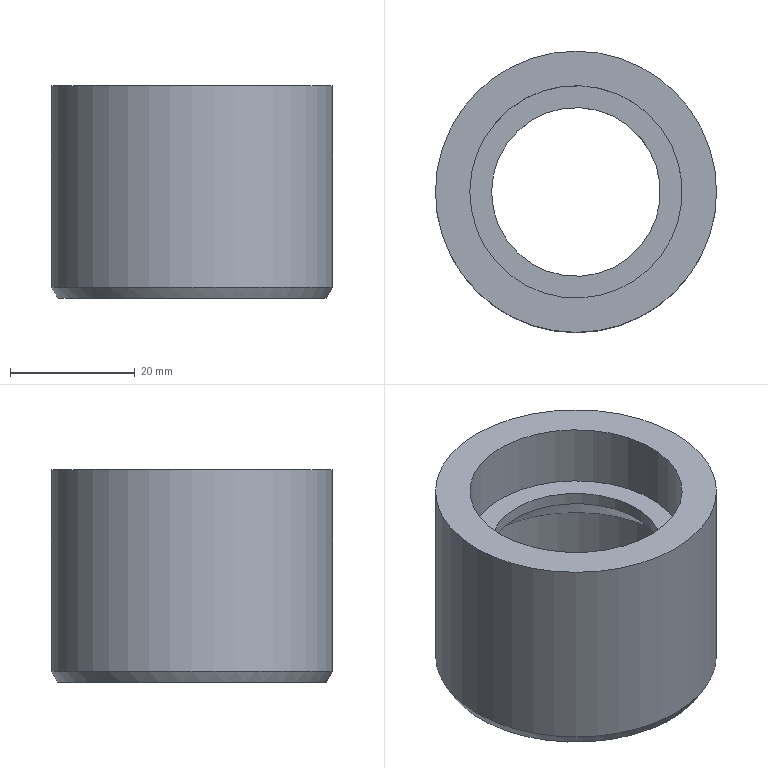Component | NX | CH3404_8_1-1 | 1 solid | 9 faces | box 45 x 45 x 34 mm | volume 19820 mm3 | cylinder 4 | plane 3 | cone 2 | commonest cylinder face diameters 45 x1 38.6 x1 27 x1 34 x1
STEP:
#1=CARTESIAN_POINT('',(0.,0.,0.));
#2=DIRECTION('',(0.,0.,1.));
#3=DIRECTION('',(1.,0.,0.));
#4=AXIS2_PLACEMENT_3D('',#1,#2,#3);
#5=CARTESIAN_POINT('',(-22.5,0.,137.));
#6=VERTEX_POINT('',#5);
#7=CARTESIAN_POINT('',(0.,0.,137.));
#8=DIRECTION('',(0.,0.,-1.));
#9=DIRECTION('',(-1.,0.,0.));
#10=AXIS2_PLACEMENT_3D('',#7,#8,#9);
#11=CIRCLE('',#10,22.5);
#12=CARTESIAN_POINT('',(0.,-17.,137.));
#13=DIRECTION('',(0.,0.,-1.));
#14=DIRECTION('',(-1.,0.,0.));
#15=AXIS2_PLACEMENT_3D('',#12,#13,#14);
#16=PLANE('',#15);
#17=CARTESIAN_POINT('',(0.,17.));
#18=DIRECTION('',(1.,0.));
#19=AXIS2_PLACEMENT_2D('',#17,#18);
#20=CIRCLE('',#19,22.5);
#21=(GEOMETRIC_REPRESENTATION_CONTEXT(2)PARAMETRIC_REPRESENTATION_CONTEXT()REPRESENTATION_CONTEXT('',''));
#22=DEFINITIONAL_REPRESENTATION('',(#20),#21);
#23=PCURVE('',#16,#22);
#24=CARTESIAN_POINT('',(0.,0.,103.));
#25=DIRECTION('',(0.,0.,-1.));
#26=DIRECTION('',(-1.,0.,0.));
#27=AXIS2_PLACEMENT_3D('',#24,#25,#26);
#28=CYLINDRICAL_SURFACE('',#27,22.5);
#29=CARTESIAN_POINT('',(0.,-34.));
#30=DIRECTION('',(1.,0.));
#31=VECTOR('',#30,1.);
#32=LINE('',#29,#31);
#33=(GEOMETRIC_REPRESENTATION_CONTEXT(2)PARAMETRIC_REPRESENTATION_CONTEXT()REPRESENTATION_CONTEXT('',''));
#34=DEFINITIONAL_REPRESENTATION('',(#32),#33);
#35=PCURVE('',#28,#34);
#36=SURFACE_CURVE('',#11,(#23,#35),.PCURVE_S1.);
#37=EDGE_CURVE('',#6,#6,#36,.T.);
#38=ORIENTED_EDGE('',*,*,#37,.F.);
#39=EDGE_LOOP('',(#38));
#40=FACE_BOUND('',#39,.T.);
#41=CARTESIAN_POINT('',(-17.,0.,137.));
#42=VERTEX_POINT('',#41);
#43=CARTESIAN_POINT('',(0.,0.,137.));
#44=DIRECTION('',(0.,0.,-1.));
#45=DIRECTION('',(-1.,0.,0.));
#46=AXIS2_PLACEMENT_3D('',#43,#44,#45);
#47=CIRCLE('',#46,17.);
#48=CARTESIAN_POINT('',(0.,17.));
#49=DIRECTION('',(1.,0.));
#50=AXIS2_PLACEMENT_2D('',#48,#49);
#51=CIRCLE('',#50,17.);
#52=(GEOMETRIC_REPRESENTATION_CONTEXT(2)PARAMETRIC_REPRESENTATION_CONTEXT()REPRESENTATION_CONTEXT('',''));
#53=DEFINITIONAL_REPRESENTATION('',(#51),#52);
#54=PCURVE('',#16,#53);
#55=CARTESIAN_POINT('',(0.,0.,103.));
#56=DIRECTION('',(0.,0.,-1.));
#57=DIRECTION('',(-1.,0.,0.));
#58=AXIS2_PLACEMENT_3D('',#55,#56,#57);
#59=CYLINDRICAL_SURFACE('',#58,17.);
#60=CARTESIAN_POINT('',(0.,-34.));
#61=DIRECTION('',(1.,0.));
#62=VECTOR('',#61,1.);
#63=LINE('',#60,#62);
#64=(GEOMETRIC_REPRESENTATION_CONTEXT(2)PARAMETRIC_REPRESENTATION_CONTEXT()REPRESENTATION_CONTEXT('',''));
#65=DEFINITIONAL_REPRESENTATION('',(#63),#64);
#66=PCURVE('',#59,#65);
#67=SURFACE_CURVE('',#47,(#54,#66),.PCURVE_S1.);
#68=EDGE_CURVE('',#42,#42,#67,.T.);
#69=ORIENTED_EDGE('',*,*,#68,.T.);
#70=EDGE_LOOP('',(#69));
#71=FACE_BOUND('',#70,.T.);
#72=ADVANCED_FACE('',(#40,#71),#16,.F.);
#73=CARTESIAN_POINT('',(22.5,0.,104.732));
#74=VERTEX_POINT('',#73);
#75=CARTESIAN_POINT('',(-22.5,0.,104.732));
#76=VERTEX_POINT('',#75);
#77=CARTESIAN_POINT('',(0.,0.,104.732));
#78=DIRECTION('',(0.,0.,1.));
#79=DIRECTION('',(1.,0.,0.));
#80=AXIS2_PLACEMENT_3D('',#77,#78,#79);
#81=CIRCLE('',#80,22.5);
#82=CARTESIAN_POINT('',(3.142,-1.732));
#83=DIRECTION('',(-1.,0.));
#84=VECTOR('',#83,1.);
#85=LINE('',#82,#84);
#86=(GEOMETRIC_REPRESENTATION_CONTEXT(2)PARAMETRIC_REPRESENTATION_CONTEXT()REPRESENTATION_CONTEXT('',''));
#87=DEFINITIONAL_REPRESENTATION('',(#85),#86);
#88=PCURVE('',#28,#87);
#89=CARTESIAN_POINT('',(0.,0.,103.));
#90=DIRECTION('',(0.,0.,1.));
#91=DIRECTION('',(1.,0.,0.));
#92=AXIS2_PLACEMENT_3D('',#89,#90,#91);
#93=CONICAL_SURFACE('',#92,21.5,0.5236);
#94=CARTESIAN_POINT('',(0.,1.732));
#95=DIRECTION('',(1.,0.));
#96=VECTOR('',#95,1.);
#97=LINE('',#94,#96);
#98=(GEOMETRIC_REPRESENTATION_CONTEXT(2)PARAMETRIC_REPRESENTATION_CONTEXT()REPRESENTATION_CONTEXT('',''));
#99=DEFINITIONAL_REPRESENTATION('',(#97),#98);
#100=PCURVE('',#93,#99);
#101=SURFACE_CURVE('',#81,(#88,#100),.PCURVE_S1.);
#102=EDGE_CURVE('',#74,#76,#101,.T.);
#103=ORIENTED_EDGE('',*,*,#102,.T.);
#104=CARTESIAN_POINT('',(-22.5,-0.,137.));
#105=CARTESIAN_POINT('',(-22.5,-0.,104.732));
#106=B_SPLINE_CURVE_WITH_KNOTS('',1,(#104,#105),.UNSPECIFIED.,.F.,.F.,(2,2),(-34.,-1.732),.PIECEWISE_BEZIER_KNOTS.);
#107=CARTESIAN_POINT('',(0.,0.));
#108=DIRECTION('',(0.,1.));
#109=VECTOR('',#108,1.);
#110=LINE('',#107,#109);
#111=(GEOMETRIC_REPRESENTATION_CONTEXT(2)PARAMETRIC_REPRESENTATION_CONTEXT()REPRESENTATION_CONTEXT('',''));
#112=DEFINITIONAL_REPRESENTATION('',(#110),#111);
#113=PCURVE('',#28,#112);
#114=CARTESIAN_POINT('',(6.283,0.));
#115=DIRECTION('',(0.,1.));
#116=VECTOR('',#115,1.);
#117=LINE('',#114,#116);
#118=(GEOMETRIC_REPRESENTATION_CONTEXT(2)PARAMETRIC_REPRESENTATION_CONTEXT()REPRESENTATION_CONTEXT('',''));
#119=DEFINITIONAL_REPRESENTATION('',(#117),#118);
#120=PCURVE('',#28,#119);
#121=SEAM_CURVE('',#106,(#113,#120),.PCURVE_S1.);
#122=EDGE_CURVE('',#6,#76,#121,.T.);
#123=ORIENTED_EDGE('',*,*,#122,.F.);
#124=ORIENTED_EDGE('',*,*,#37,.T.);
#125=ORIENTED_EDGE('',*,*,#122,.T.);
#126=CARTESIAN_POINT('',(0.,0.,104.732));
#127=DIRECTION('',(0.,0.,1.));
#128=DIRECTION('',(1.,0.,0.));
#129=AXIS2_PLACEMENT_3D('',#126,#127,#128);
#130=CIRCLE('',#129,22.5);
#131=CARTESIAN_POINT('',(9.425,-1.732));
#132=DIRECTION('',(-1.,0.));
#133=VECTOR('',#132,1.);
#134=LINE('',#131,#133);
#135=(GEOMETRIC_REPRESENTATION_CONTEXT(2)PARAMETRIC_REPRESENTATION_CONTEXT()REPRESENTATION_CONTEXT('',''));
#136=DEFINITIONAL_REPRESENTATION('',(#134),#135);
#137=PCURVE('',#28,#136);
#138=CARTESIAN_POINT('',(0.,1.732));
#139=DIRECTION('',(1.,0.));
#140=VECTOR('',#139,1.);
#141=LINE('',#138,#140);
#142=(GEOMETRIC_REPRESENTATION_CONTEXT(2)PARAMETRIC_REPRESENTATION_CONTEXT()REPRESENTATION_CONTEXT('',''));
#143=DEFINITIONAL_REPRESENTATION('',(#141),#142);
#144=PCURVE('',#93,#143);
#145=SURFACE_CURVE('',#130,(#137,#144),.PCURVE_S1.);
#146=EDGE_CURVE('',#76,#74,#145,.T.);
#147=ORIENTED_EDGE('',*,*,#146,.T.);
#148=EDGE_LOOP('',(#103,#123,#124,#125,#147));
#149=FACE_BOUND('',#148,.T.);
#150=ADVANCED_FACE('',(#149),#28,.T.);
#151=CARTESIAN_POINT('',(21.5,0.,103.));
#152=VERTEX_POINT('',#151);
#153=CARTESIAN_POINT('',(0.,0.,103.));
#154=DIRECTION('',(0.,0.,-1.));
#155=DIRECTION('',(1.,0.,0.));
#156=AXIS2_PLACEMENT_3D('',#153,#154,#155);
#157=CIRCLE('',#156,21.5);
#158=CARTESIAN_POINT('',(0.,-22.5,103.));
#159=DIRECTION('',(0.,0.,1.));
#160=DIRECTION('',(1.,0.,0.));
#161=AXIS2_PLACEMENT_3D('',#158,#159,#160);
#162=PLANE('',#161);
#163=CARTESIAN_POINT('',(21.5,22.5));
#164=CARTESIAN_POINT('',(21.5,-14.739));
#165=CARTESIAN_POINT('',(-10.75,3.88));
#166=CARTESIAN_POINT('',(-43.,22.5));
#167=CARTESIAN_POINT('',(-10.75,41.12));
#168=CARTESIAN_POINT('',(21.5,59.739));
#169=CARTESIAN_POINT('',(21.5,22.5));
#170=(BOUNDED_CURVE()B_SPLINE_CURVE(2,(#163,#164,#165,#166,#167,#168,#169),.UNSPECIFIED.,.T.,.F.)B_SPLINE_CURVE_WITH_KNOTS((1,2,2,2,2,1),(-2.094,0.,2.094,4.189,6.283,8.378),.UNSPECIFIED.)CURVE()GEOMETRIC_REPRESENTATION_ITEM()RATIONAL_B_SPLINE_CURVE((1.,0.5,1.,0.5,1.,0.5,1.))REPRESENTATION_ITEM(''));
#171=(GEOMETRIC_REPRESENTATION_CONTEXT(2)PARAMETRIC_REPRESENTATION_CONTEXT()REPRESENTATION_CONTEXT('',''));
#172=DEFINITIONAL_REPRESENTATION('',(#170),#171);
#173=PCURVE('',#162,#172);
#174=CARTESIAN_POINT('',(6.283,0.));
#175=DIRECTION('',(-1.,0.));
#176=VECTOR('',#175,1.);
#177=LINE('',#174,#176);
#178=(GEOMETRIC_REPRESENTATION_CONTEXT(2)PARAMETRIC_REPRESENTATION_CONTEXT()REPRESENTATION_CONTEXT('',''));
#179=DEFINITIONAL_REPRESENTATION('',(#177),#178);
#180=PCURVE('',#93,#179);
#181=SURFACE_CURVE('',#157,(#173,#180),.PCURVE_S1.);
#182=EDGE_CURVE('',#152,#152,#181,.T.);
#183=ORIENTED_EDGE('',*,*,#182,.T.);
#184=EDGE_LOOP('',(#183));
#185=FACE_BOUND('',#184,.T.);
#186=CARTESIAN_POINT('',(-19.3,0.,103.));
#187=VERTEX_POINT('',#186);
#188=CARTESIAN_POINT('',(0.,0.,103.));
#189=DIRECTION('',(0.,0.,-1.));
#190=DIRECTION('',(-1.,0.,0.));
#191=AXIS2_PLACEMENT_3D('',#188,#189,#190);
#192=CIRCLE('',#191,19.3);
#193=CARTESIAN_POINT('',(-19.3,22.5));
#194=CARTESIAN_POINT('',(-19.3,55.929));
#195=CARTESIAN_POINT('',(9.65,39.214));
#196=CARTESIAN_POINT('',(38.6,22.5));
#197=CARTESIAN_POINT('',(9.65,5.786));
#198=CARTESIAN_POINT('',(-19.3,-10.929));
#199=CARTESIAN_POINT('',(-19.3,22.5));
#200=(BOUNDED_CURVE()B_SPLINE_CURVE(2,(#193,#194,#195,#196,#197,#198,#199),.UNSPECIFIED.,.T.,.F.)B_SPLINE_CURVE_WITH_KNOTS((1,2,2,2,2,1),(-2.094,0.,2.094,4.189,6.283,8.378),.UNSPECIFIED.)CURVE()GEOMETRIC_REPRESENTATION_ITEM()RATIONAL_B_SPLINE_CURVE((1.,0.5,1.,0.5,1.,0.5,1.))REPRESENTATION_ITEM(''));
#201=(GEOMETRIC_REPRESENTATION_CONTEXT(2)PARAMETRIC_REPRESENTATION_CONTEXT()REPRESENTATION_CONTEXT('',''));
#202=DEFINITIONAL_REPRESENTATION('',(#200),#201);
#203=PCURVE('',#162,#202);
#204=CARTESIAN_POINT('',(0.,0.,103.));
#205=DIRECTION('',(0.,0.,-1.));
#206=DIRECTION('',(-1.,0.,0.));
#207=AXIS2_PLACEMENT_3D('',#204,#205,#206);
#208=CYLINDRICAL_SURFACE('',#207,19.3);
#209=CARTESIAN_POINT('',(0.,0.));
#210=DIRECTION('',(1.,0.));
#211=VECTOR('',#210,1.);
#212=LINE('',#209,#211);
#213=(GEOMETRIC_REPRESENTATION_CONTEXT(2)PARAMETRIC_REPRESENTATION_CONTEXT()REPRESENTATION_CONTEXT('',''));
#214=DEFINITIONAL_REPRESENTATION('',(#212),#213);
#215=PCURVE('',#208,#214);
#216=SURFACE_CURVE('',#192,(#203,#215),.PCURVE_S1.);
#217=EDGE_CURVE('',#187,#187,#216,.T.);
#218=ORIENTED_EDGE('',*,*,#217,.F.);
#219=EDGE_LOOP('',(#218));
#220=FACE_BOUND('',#219,.T.);
#221=ADVANCED_FACE('',(#185,#220),#162,.F.);
#222=CARTESIAN_POINT('',(-19.3,0.,119.2));
#223=VERTEX_POINT('',#222);
#224=CARTESIAN_POINT('',(0.,0.,119.2));
#225=DIRECTION('',(0.,0.,-1.));
#226=DIRECTION('',(-1.,0.,0.));
#227=AXIS2_PLACEMENT_3D('',#224,#225,#226);
#228=CIRCLE('',#227,19.3);
#229=CARTESIAN_POINT('',(0.,-16.2));
#230=DIRECTION('',(1.,0.));
#231=VECTOR('',#230,1.);
#232=LINE('',#229,#231);
#233=(GEOMETRIC_REPRESENTATION_CONTEXT(2)PARAMETRIC_REPRESENTATION_CONTEXT()REPRESENTATION_CONTEXT('',''));
#234=DEFINITIONAL_REPRESENTATION('',(#232),#233);
#235=PCURVE('',#208,#234);
#236=CARTESIAN_POINT('',(0.,0.,119.2));
#237=DIRECTION('',(0.,0.,-1.));
#238=DIRECTION('',(-1.,0.,0.));
#239=AXIS2_PLACEMENT_3D('',#236,#237,#238);
#240=CONICAL_SURFACE('',#239,19.3,0.7854);
#241=CARTESIAN_POINT('',(0.,0.));
#242=DIRECTION('',(1.,0.));
#243=VECTOR('',#242,1.);
#244=LINE('',#241,#243);
#245=(GEOMETRIC_REPRESENTATION_CONTEXT(2)PARAMETRIC_REPRESENTATION_CONTEXT()REPRESENTATION_CONTEXT('',''));
#246=DEFINITIONAL_REPRESENTATION('',(#244),#245);
#247=PCURVE('',#240,#246);
#248=SURFACE_CURVE('',#228,(#235,#247),.PCURVE_S1.);
#249=EDGE_CURVE('',#223,#223,#248,.T.);
#250=ORIENTED_EDGE('',*,*,#249,.T.);
#251=CARTESIAN_POINT('',(-19.3,0.,119.2));
#252=CARTESIAN_POINT('',(-19.3,0.,103.));
#253=B_SPLINE_CURVE_WITH_KNOTS('',1,(#251,#252),.UNSPECIFIED.,.F.,.F.,(2,2),(-16.2,0.),.PIECEWISE_BEZIER_KNOTS.);
#254=CARTESIAN_POINT('',(6.283,0.));
#255=DIRECTION('',(0.,1.));
#256=VECTOR('',#255,1.);
#257=LINE('',#254,#256);
#258=(GEOMETRIC_REPRESENTATION_CONTEXT(2)PARAMETRIC_REPRESENTATION_CONTEXT()REPRESENTATION_CONTEXT('',''));
#259=DEFINITIONAL_REPRESENTATION('',(#257),#258);
#260=PCURVE('',#208,#259);
#261=CARTESIAN_POINT('',(0.,0.));
#262=DIRECTION('',(0.,1.));
#263=VECTOR('',#262,1.);
#264=LINE('',#261,#263);
#265=(GEOMETRIC_REPRESENTATION_CONTEXT(2)PARAMETRIC_REPRESENTATION_CONTEXT()REPRESENTATION_CONTEXT('',''));
#266=DEFINITIONAL_REPRESENTATION('',(#264),#265);
#267=PCURVE('',#208,#266);
#268=SEAM_CURVE('',#253,(#260,#267),.PCURVE_S1.);
#269=EDGE_CURVE('',#223,#187,#268,.T.);
#270=ORIENTED_EDGE('',*,*,#269,.T.);
#271=ORIENTED_EDGE('',*,*,#217,.F.);
#272=ORIENTED_EDGE('',*,*,#269,.F.);
#273=EDGE_LOOP('',(#250,#270,#271,#272));
#274=FACE_BOUND('',#273,.F.);
#275=ADVANCED_FACE('',(#274),#208,.F.);
#276=CARTESIAN_POINT('',(-13.5,0.,125.));
#277=VERTEX_POINT('',#276);
#278=CARTESIAN_POINT('',(0.,0.,125.));
#279=DIRECTION('',(0.,0.,-1.));
#280=DIRECTION('',(-1.,0.,0.));
#281=AXIS2_PLACEMENT_3D('',#278,#279,#280);
#282=CIRCLE('',#281,13.5);
#283=CARTESIAN_POINT('',(0.,-5.8));
#284=DIRECTION('',(1.,0.));
#285=VECTOR('',#284,1.);
#286=LINE('',#283,#285);
#287=(GEOMETRIC_REPRESENTATION_CONTEXT(2)PARAMETRIC_REPRESENTATION_CONTEXT()REPRESENTATION_CONTEXT('',''));
#288=DEFINITIONAL_REPRESENTATION('',(#286),#287);
#289=PCURVE('',#240,#288);
#290=CARTESIAN_POINT('',(0.,0.,103.));
#291=DIRECTION('',(0.,0.,-1.));
#292=DIRECTION('',(-1.,0.,0.));
#293=AXIS2_PLACEMENT_3D('',#290,#291,#292);
#294=CYLINDRICAL_SURFACE('',#293,13.5);
#295=CARTESIAN_POINT('',(0.,-22.));
#296=DIRECTION('',(1.,0.));
#297=VECTOR('',#296,1.);
#298=LINE('',#295,#297);
#299=(GEOMETRIC_REPRESENTATION_CONTEXT(2)PARAMETRIC_REPRESENTATION_CONTEXT()REPRESENTATION_CONTEXT('',''));
#300=DEFINITIONAL_REPRESENTATION('',(#298),#299);
#301=PCURVE('',#294,#300);
#302=SURFACE_CURVE('',#282,(#289,#301),.PCURVE_S1.);
#303=EDGE_CURVE('',#277,#277,#302,.T.);
#304=ORIENTED_EDGE('',*,*,#303,.T.);
#305=CARTESIAN_POINT('',(-13.5,0.,125.));
#306=CARTESIAN_POINT('',(-19.3,0.,119.2));
#307=B_SPLINE_CURVE_WITH_KNOTS('',1,(#305,#306),.UNSPECIFIED.,.F.,.F.,(2,2),(-8.202,0.),.PIECEWISE_BEZIER_KNOTS.);
#308=CARTESIAN_POINT('',(6.283,0.));
#309=DIRECTION('',(0.,1.));
#310=VECTOR('',#309,1.);
#311=LINE('',#308,#310);
#312=(GEOMETRIC_REPRESENTATION_CONTEXT(2)PARAMETRIC_REPRESENTATION_CONTEXT()REPRESENTATION_CONTEXT('',''));
#313=DEFINITIONAL_REPRESENTATION('',(#311),#312);
#314=PCURVE('',#240,#313);
#315=CARTESIAN_POINT('',(0.,0.));
#316=DIRECTION('',(0.,1.));
#317=VECTOR('',#316,1.);
#318=LINE('',#315,#317);
#319=(GEOMETRIC_REPRESENTATION_CONTEXT(2)PARAMETRIC_REPRESENTATION_CONTEXT()REPRESENTATION_CONTEXT('',''));
#320=DEFINITIONAL_REPRESENTATION('',(#318),#319);
#321=PCURVE('',#240,#320);
#322=SEAM_CURVE('',#307,(#314,#321),.PCURVE_S1.);
#323=EDGE_CURVE('',#277,#223,#322,.T.);
#324=ORIENTED_EDGE('',*,*,#323,.T.);
#325=ORIENTED_EDGE('',*,*,#249,.F.);
#326=ORIENTED_EDGE('',*,*,#323,.F.);
#327=EDGE_LOOP('',(#304,#324,#325,#326));
#328=FACE_BOUND('',#327,.F.);
#329=ADVANCED_FACE('',(#328),#240,.F.);
#330=CARTESIAN_POINT('',(-13.5,0.,127.));
#331=VERTEX_POINT('',#330);
#332=CARTESIAN_POINT('',(0.,0.,127.));
#333=DIRECTION('',(0.,0.,-1.));
#334=DIRECTION('',(-1.,0.,0.));
#335=AXIS2_PLACEMENT_3D('',#332,#333,#334);
#336=CIRCLE('',#335,13.5);
#337=CARTESIAN_POINT('',(0.,-24.));
#338=DIRECTION('',(1.,0.));
#339=VECTOR('',#338,1.);
#340=LINE('',#337,#339);
#341=(GEOMETRIC_REPRESENTATION_CONTEXT(2)PARAMETRIC_REPRESENTATION_CONTEXT()REPRESENTATION_CONTEXT('',''));
#342=DEFINITIONAL_REPRESENTATION('',(#340),#341);
#343=PCURVE('',#294,#342);
#344=CARTESIAN_POINT('',(0.,-13.5,127.));
#345=DIRECTION('',(0.,0.,-1.));
#346=DIRECTION('',(-1.,0.,0.));
#347=AXIS2_PLACEMENT_3D('',#344,#345,#346);
#348=PLANE('',#347);
#349=CARTESIAN_POINT('',(0.,13.5));
#350=DIRECTION('',(1.,0.));
#351=AXIS2_PLACEMENT_2D('',#349,#350);
#352=CIRCLE('',#351,13.5);
#353=(GEOMETRIC_REPRESENTATION_CONTEXT(2)PARAMETRIC_REPRESENTATION_CONTEXT()REPRESENTATION_CONTEXT('',''));
#354=DEFINITIONAL_REPRESENTATION('',(#352),#353);
#355=PCURVE('',#348,#354);
#356=SURFACE_CURVE('',#336,(#343,#355),.PCURVE_S1.);
#357=EDGE_CURVE('',#331,#331,#356,.T.);
#358=ORIENTED_EDGE('',*,*,#357,.T.);
#359=CARTESIAN_POINT('',(-13.5,0.,127.));
#360=CARTESIAN_POINT('',(-13.5,0.,125.));
#361=B_SPLINE_CURVE_WITH_KNOTS('',1,(#359,#360),.UNSPECIFIED.,.F.,.F.,(2,2),(-24.,-22.),.PIECEWISE_BEZIER_KNOTS.);
#362=CARTESIAN_POINT('',(6.283,0.));
#363=DIRECTION('',(0.,1.));
#364=VECTOR('',#363,1.);
#365=LINE('',#362,#364);
#366=(GEOMETRIC_REPRESENTATION_CONTEXT(2)PARAMETRIC_REPRESENTATION_CONTEXT()REPRESENTATION_CONTEXT('',''));
#367=DEFINITIONAL_REPRESENTATION('',(#365),#366);
#368=PCURVE('',#294,#367);
#369=CARTESIAN_POINT('',(0.,0.));
#370=DIRECTION('',(0.,1.));
#371=VECTOR('',#370,1.);
#372=LINE('',#369,#371);
#373=(GEOMETRIC_REPRESENTATION_CONTEXT(2)PARAMETRIC_REPRESENTATION_CONTEXT()REPRESENTATION_CONTEXT('',''));
#374=DEFINITIONAL_REPRESENTATION('',(#372),#373);
#375=PCURVE('',#294,#374);
#376=SEAM_CURVE('',#361,(#368,#375),.PCURVE_S1.);
#377=EDGE_CURVE('',#331,#277,#376,.T.);
#378=ORIENTED_EDGE('',*,*,#377,.T.);
#379=ORIENTED_EDGE('',*,*,#303,.F.);
#380=ORIENTED_EDGE('',*,*,#377,.F.);
#381=EDGE_LOOP('',(#358,#378,#379,#380));
#382=FACE_BOUND('',#381,.F.);
#383=ADVANCED_FACE('',(#382),#294,.F.);
#384=CARTESIAN_POINT('',(-17.,0.,127.));
#385=VERTEX_POINT('',#384);
#386=CARTESIAN_POINT('',(0.,0.,127.));
#387=DIRECTION('',(0.,0.,-1.));
#388=DIRECTION('',(-1.,0.,0.));
#389=AXIS2_PLACEMENT_3D('',#386,#387,#388);
#390=CIRCLE('',#389,17.);
#391=CARTESIAN_POINT('',(0.,13.5));
#392=DIRECTION('',(1.,0.));
#393=AXIS2_PLACEMENT_2D('',#391,#392);
#394=CIRCLE('',#393,17.);
#395=(GEOMETRIC_REPRESENTATION_CONTEXT(2)PARAMETRIC_REPRESENTATION_CONTEXT()REPRESENTATION_CONTEXT('',''));
#396=DEFINITIONAL_REPRESENTATION('',(#394),#395);
#397=PCURVE('',#348,#396);
#398=CARTESIAN_POINT('',(0.,-24.));
#399=DIRECTION('',(1.,0.));
#400=VECTOR('',#399,1.);
#401=LINE('',#398,#400);
#402=(GEOMETRIC_REPRESENTATION_CONTEXT(2)PARAMETRIC_REPRESENTATION_CONTEXT()REPRESENTATION_CONTEXT('',''));
#403=DEFINITIONAL_REPRESENTATION('',(#401),#402);
#404=PCURVE('',#59,#403);
#405=SURFACE_CURVE('',#390,(#397,#404),.PCURVE_S1.);
#406=EDGE_CURVE('',#385,#385,#405,.T.);
#407=ORIENTED_EDGE('',*,*,#406,.F.);
#408=EDGE_LOOP('',(#407));
#409=FACE_BOUND('',#408,.T.);
#410=ORIENTED_EDGE('',*,*,#357,.T.);
#411=EDGE_LOOP('',(#410));
#412=FACE_BOUND('',#411,.T.);
#413=ADVANCED_FACE('',(#409,#412),#348,.F.);
#414=ORIENTED_EDGE('',*,*,#68,.T.);
#415=CARTESIAN_POINT('',(-17.,0.,137.));
#416=CARTESIAN_POINT('',(-17.,0.,127.));
#417=B_SPLINE_CURVE_WITH_KNOTS('',1,(#415,#416),.UNSPECIFIED.,.F.,.F.,(2,2),(-34.,-24.),.PIECEWISE_BEZIER_KNOTS.);
#418=CARTESIAN_POINT('',(6.283,0.));
#419=DIRECTION('',(0.,1.));
#420=VECTOR('',#419,1.);
#421=LINE('',#418,#420);
#422=(GEOMETRIC_REPRESENTATION_CONTEXT(2)PARAMETRIC_REPRESENTATION_CONTEXT()REPRESENTATION_CONTEXT('',''));
#423=DEFINITIONAL_REPRESENTATION('',(#421),#422);
#424=PCURVE('',#59,#423);
#425=CARTESIAN_POINT('',(0.,0.));
#426=DIRECTION('',(0.,1.));
#427=VECTOR('',#426,1.);
#428=LINE('',#425,#427);
#429=(GEOMETRIC_REPRESENTATION_CONTEXT(2)PARAMETRIC_REPRESENTATION_CONTEXT()REPRESENTATION_CONTEXT('',''));
#430=DEFINITIONAL_REPRESENTATION('',(#428),#429);
#431=PCURVE('',#59,#430);
#432=SEAM_CURVE('',#417,(#424,#431),.PCURVE_S1.);
#433=EDGE_CURVE('',#42,#385,#432,.T.);
#434=ORIENTED_EDGE('',*,*,#433,.T.);
#435=ORIENTED_EDGE('',*,*,#406,.F.);
#436=ORIENTED_EDGE('',*,*,#433,.F.);
#437=EDGE_LOOP('',(#414,#434,#435,#436));
#438=FACE_BOUND('',#437,.F.);
#439=ADVANCED_FACE('',(#438),#59,.F.);
#440=ORIENTED_EDGE('',*,*,#102,.F.);
#441=CARTESIAN_POINT('',(21.5,-0.,103.));
#442=CARTESIAN_POINT('',(22.5,-0.,104.732));
#443=B_SPLINE_CURVE_WITH_KNOTS('',1,(#441,#442),.UNSPECIFIED.,.F.,.F.,(2,2),(0.,2.),.PIECEWISE_BEZIER_KNOTS.);
#444=CARTESIAN_POINT('',(0.,0.));
#445=DIRECTION('',(0.,1.));
#446=VECTOR('',#445,1.);
#447=LINE('',#444,#446);
#448=(GEOMETRIC_REPRESENTATION_CONTEXT(2)PARAMETRIC_REPRESENTATION_CONTEXT()REPRESENTATION_CONTEXT('',''));
#449=DEFINITIONAL_REPRESENTATION('',(#447),#448);
#450=PCURVE('',#93,#449);
#451=CARTESIAN_POINT('',(6.283,0.));
#452=DIRECTION('',(0.,1.));
#453=VECTOR('',#452,1.);
#454=LINE('',#451,#453);
#455=(GEOMETRIC_REPRESENTATION_CONTEXT(2)PARAMETRIC_REPRESENTATION_CONTEXT()REPRESENTATION_CONTEXT('',''));
#456=DEFINITIONAL_REPRESENTATION('',(#454),#455);
#457=PCURVE('',#93,#456);
#458=SEAM_CURVE('',#443,(#450,#457),.PCURVE_S1.);
#459=EDGE_CURVE('',#152,#74,#458,.T.);
#460=ORIENTED_EDGE('',*,*,#459,.F.);
#461=ORIENTED_EDGE('',*,*,#182,.F.);
#462=ORIENTED_EDGE('',*,*,#459,.T.);
#463=ORIENTED_EDGE('',*,*,#146,.F.);
#464=EDGE_LOOP('',(#440,#460,#461,#462,#463));
#465=FACE_BOUND('',#464,.T.);
#466=ADVANCED_FACE('',(#465),#93,.T.);
#467=CLOSED_SHELL('',(#72,#150,#221,#275,#329,#383,#413,#439,#466));
#468=MANIFOLD_SOLID_BREP('',#467);
#469=(LENGTH_UNIT()NAMED_UNIT(*)SI_UNIT(.MILLI.,.METRE.));
#470=UNCERTAINTY_MEASURE_WITH_UNIT(LENGTH_MEASURE(0.00001),#469,'','');
#471=(NAMED_UNIT(*)PLANE_ANGLE_UNIT()SI_UNIT($,.RADIAN.));
#472=(NAMED_UNIT(*)SI_UNIT($,.STERADIAN.)SOLID_ANGLE_UNIT());
#473=(GEOMETRIC_REPRESENTATION_CONTEXT(3)GLOBAL_UNCERTAINTY_ASSIGNED_CONTEXT((#470))GLOBAL_UNIT_ASSIGNED_CONTEXT((#469,#471,#472))REPRESENTATION_CONTEXT('',''));
#474=ADVANCED_BREP_SHAPE_REPRESENTATION('',(#4,#468),#473);